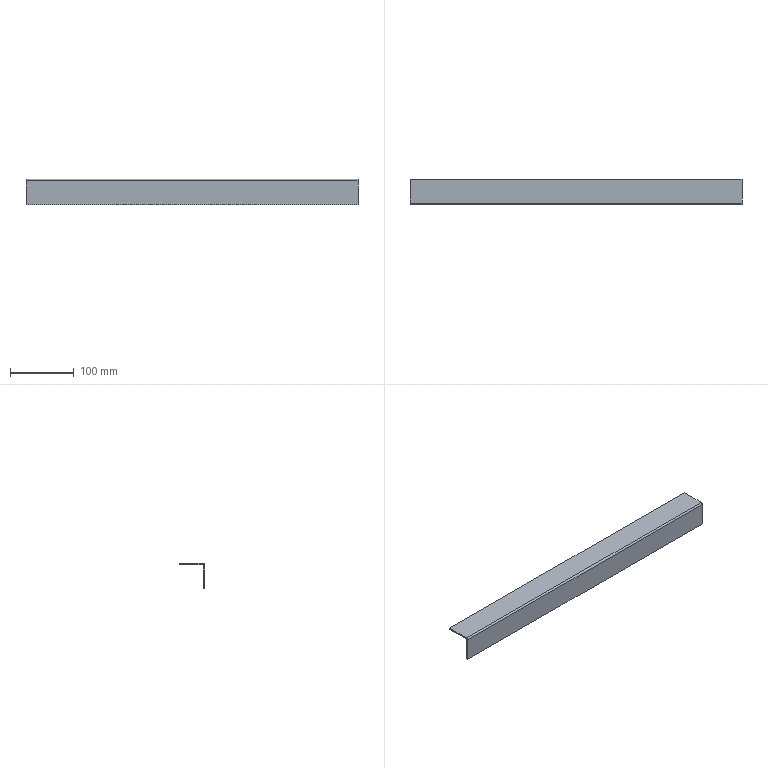Component | SolidWorks | BaseBracketAssembly-1_BaseBracketWidth-7 | 1 solid | 14 faces | box 520 x 40 x 40 mm | volume 80450 mm3 | plane 12 | cylinder 2 | commonest cylinder face diameters 5 x1 1 x1 | material 2.0mm Cold Rolled Plate
STEP:
#1=CARTESIAN_POINT('',(-11.983,-50.005,37.594));
#2=VERTEX_POINT('',#1);
#3=CARTESIAN_POINT('',(-11.983,-49.926,37.594));
#4=VERTEX_POINT('',#3);
#5=CARTESIAN_POINT('',(-11.983,-50.005,37.594));
#6=DIRECTION('',(0.,1.,0.));
#7=VECTOR('',#6,39.37);
#8=LINE('',#5,#7);
#9=EDGE_CURVE('',#2,#4,#8,.T.);
#10=ORIENTED_EDGE('',*,*,#9,.F.);
#11=CARTESIAN_POINT('',(-11.983,-49.907,37.692));
#12=VERTEX_POINT('',#11);
#13=CARTESIAN_POINT('',(-11.983,-49.907,37.594));
#14=DIRECTION('',(1.,-0.,-0.));
#15=DIRECTION('',(0.,1.,0.));
#16=AXIS2_PLACEMENT_3D('',#13,#14,#15);
#17=CIRCLE('',#16,0.09843);
#18=EDGE_CURVE('',#12,#2,#17,.T.);
#19=ORIENTED_EDGE('',*,*,#18,.F.);
#20=CARTESIAN_POINT('',(-11.983,-49.907,37.614));
#21=VERTEX_POINT('',#20);
#22=CARTESIAN_POINT('',(-11.983,-49.907,37.614));
#23=DIRECTION('',(0.,-0.,1.));
#24=VECTOR('',#23,39.37);
#25=LINE('',#22,#24);
#26=EDGE_CURVE('',#21,#12,#25,.T.);
#27=ORIENTED_EDGE('',*,*,#26,.F.);
#28=CARTESIAN_POINT('',(-11.983,-49.907,37.594));
#29=DIRECTION('',(1.,-0.,-0.));
#30=DIRECTION('',(0.,1.,0.));
#31=AXIS2_PLACEMENT_3D('',#28,#29,#30);
#32=CIRCLE('',#31,0.01969);
#33=EDGE_CURVE('',#21,#4,#32,.T.);
#34=ORIENTED_EDGE('',*,*,#33,.T.);
#35=EDGE_LOOP('',(#10,#19,#27,#34));
#36=FACE_OUTER_BOUND('',#35,.T.);
#37=CARTESIAN_POINT('',(-11.983,-50.005,37.594));
#38=DIRECTION('',(-1.,0.,0.));
#39=DIRECTION('',(0.,1.,0.));
#40=AXIS2_PLACEMENT_3D('',#37,#38,#39);
#41=PLANE('',#40);
#42=ADVANCED_FACE('',(#36),#41,.T.);
#43=CARTESIAN_POINT('',(-11.983,-50.005,36.118));
#44=VERTEX_POINT('',#43);
#45=CARTESIAN_POINT('',(-11.983,-50.005,36.118));
#46=DIRECTION('',(-0.,0.,-1.));
#47=VECTOR('',#46,39.37);
#48=LINE('',#45,#47);
#49=EDGE_CURVE('',#2,#44,#48,.T.);
#50=ORIENTED_EDGE('',*,*,#49,.F.);
#51=ORIENTED_EDGE('',*,*,#9,.T.);
#52=CARTESIAN_POINT('',(-11.983,-49.926,36.118));
#53=VERTEX_POINT('',#52);
#54=CARTESIAN_POINT('',(-11.983,-49.926,36.118));
#55=DIRECTION('',(-0.,0.,-1.));
#56=VECTOR('',#55,39.37);
#57=LINE('',#54,#56);
#58=EDGE_CURVE('',#4,#53,#57,.T.);
#59=ORIENTED_EDGE('',*,*,#58,.T.);
#60=CARTESIAN_POINT('',(-11.983,-50.005,36.118));
#61=DIRECTION('',(0.,1.,0.));
#62=VECTOR('',#61,39.37);
#63=LINE('',#60,#62);
#64=EDGE_CURVE('',#44,#53,#63,.T.);
#65=ORIENTED_EDGE('',*,*,#64,.F.);
#66=EDGE_LOOP('',(#50,#51,#59,#65));
#67=FACE_OUTER_BOUND('',#66,.T.);
#68=CARTESIAN_POINT('',(-11.983,-49.907,37.614));
#69=DIRECTION('',(-1.,0.,0.));
#70=DIRECTION('',(0.,1.,0.));
#71=AXIS2_PLACEMENT_3D('',#68,#69,#70);
#72=PLANE('',#71);
#73=ADVANCED_FACE('',(#67),#72,.T.);
#74=CARTESIAN_POINT('',(8.49,-49.907,37.692));
#75=VERTEX_POINT('',#74);
#76=CARTESIAN_POINT('',(8.49,-49.907,37.614));
#77=VERTEX_POINT('',#76);
#78=CARTESIAN_POINT('',(8.49,-49.907,37.692));
#79=DIRECTION('',(-0.,0.,-1.));
#80=VECTOR('',#79,39.37);
#81=LINE('',#78,#80);
#82=EDGE_CURVE('',#75,#77,#81,.T.);
#83=ORIENTED_EDGE('',*,*,#82,.F.);
#84=CARTESIAN_POINT('',(8.49,-50.005,37.594));
#85=VERTEX_POINT('',#84);
#86=CARTESIAN_POINT('',(8.49,-49.907,37.594));
#87=DIRECTION('',(1.,-0.,-0.));
#88=DIRECTION('',(0.,1.,0.));
#89=AXIS2_PLACEMENT_3D('',#86,#87,#88);
#90=CIRCLE('',#89,0.09843);
#91=EDGE_CURVE('',#75,#85,#90,.T.);
#92=ORIENTED_EDGE('',*,*,#91,.T.);
#93=CARTESIAN_POINT('',(8.49,-49.926,37.594));
#94=VERTEX_POINT('',#93);
#95=CARTESIAN_POINT('',(8.49,-49.926,37.594));
#96=DIRECTION('',(-0.,-1.,-0.));
#97=VECTOR('',#96,39.37);
#98=LINE('',#95,#97);
#99=EDGE_CURVE('',#94,#85,#98,.T.);
#100=ORIENTED_EDGE('',*,*,#99,.F.);
#101=CARTESIAN_POINT('',(8.49,-49.907,37.594));
#102=DIRECTION('',(1.,-0.,-0.));
#103=DIRECTION('',(0.,1.,0.));
#104=AXIS2_PLACEMENT_3D('',#101,#102,#103);
#105=CIRCLE('',#104,0.01969);
#106=EDGE_CURVE('',#77,#94,#105,.T.);
#107=ORIENTED_EDGE('',*,*,#106,.F.);
#108=EDGE_LOOP('',(#83,#92,#100,#107));
#109=FACE_OUTER_BOUND('',#108,.T.);
#110=CARTESIAN_POINT('',(8.49,-49.907,37.692));
#111=DIRECTION('',(1.,-0.,-0.));
#112=DIRECTION('',(-0.,-1.,-0.));
#113=AXIS2_PLACEMENT_3D('',#110,#111,#112);
#114=PLANE('',#113);
#115=ADVANCED_FACE('',(#109),#114,.T.);
#116=CARTESIAN_POINT('',(8.49,-48.43,37.692));
#117=VERTEX_POINT('',#116);
#118=CARTESIAN_POINT('',(8.49,-50.005,37.692));
#119=DIRECTION('',(-0.,-1.,-0.));
#120=VECTOR('',#119,39.37);
#121=LINE('',#118,#120);
#122=EDGE_CURVE('',#117,#75,#121,.T.);
#123=ORIENTED_EDGE('',*,*,#122,.T.);
#124=ORIENTED_EDGE('',*,*,#82,.T.);
#125=CARTESIAN_POINT('',(8.49,-48.43,37.614));
#126=VERTEX_POINT('',#125);
#127=CARTESIAN_POINT('',(8.49,-50.005,37.614));
#128=DIRECTION('',(-0.,-1.,-0.));
#129=VECTOR('',#128,39.37);
#130=LINE('',#127,#129);
#131=EDGE_CURVE('',#126,#77,#130,.T.);
#132=ORIENTED_EDGE('',*,*,#131,.F.);
#133=CARTESIAN_POINT('',(8.49,-48.43,37.614));
#134=DIRECTION('',(0.,-0.,1.));
#135=VECTOR('',#134,39.37);
#136=LINE('',#133,#135);
#137=EDGE_CURVE('',#126,#117,#136,.T.);
#138=ORIENTED_EDGE('',*,*,#137,.T.);
#139=EDGE_LOOP('',(#123,#124,#132,#138));
#140=FACE_OUTER_BOUND('',#139,.T.);
#141=CARTESIAN_POINT('',(8.49,-49.926,37.594));
#142=DIRECTION('',(1.,-0.,-0.));
#143=DIRECTION('',(-0.,-1.,-0.));
#144=AXIS2_PLACEMENT_3D('',#141,#142,#143);
#145=PLANE('',#144);
#146=ADVANCED_FACE('',(#140),#145,.T.);
#147=CARTESIAN_POINT('',(8.49,-49.926,36.118));
#148=VERTEX_POINT('',#147);
#149=CARTESIAN_POINT('',(8.49,-49.926,36.118));
#150=DIRECTION('',(-0.,0.,-1.));
#151=VECTOR('',#150,39.37);
#152=LINE('',#149,#151);
#153=EDGE_CURVE('',#94,#148,#152,.T.);
#154=ORIENTED_EDGE('',*,*,#153,.T.);
#155=CARTESIAN_POINT('',(-11.983,-49.926,36.118));
#156=DIRECTION('',(1.,-0.,-0.));
#157=VECTOR('',#156,39.37);
#158=LINE('',#155,#157);
#159=EDGE_CURVE('',#53,#148,#158,.T.);
#160=ORIENTED_EDGE('',*,*,#159,.F.);
#161=ORIENTED_EDGE('',*,*,#58,.F.);
#162=CARTESIAN_POINT('',(-11.983,-49.926,37.594));
#163=DIRECTION('',(1.,-0.,-0.));
#164=VECTOR('',#163,39.37);
#165=LINE('',#162,#164);
#166=EDGE_CURVE('',#4,#94,#165,.T.);
#167=ORIENTED_EDGE('',*,*,#166,.T.);
#168=EDGE_LOOP('',(#154,#160,#161,#167));
#169=FACE_OUTER_BOUND('',#168,.T.);
#170=CARTESIAN_POINT('',(-11.983,-49.926,36.118));
#171=DIRECTION('',(-0.,-1.,-0.));
#172=DIRECTION('',(-1.,0.,0.));
#173=AXIS2_PLACEMENT_3D('',#170,#171,#172);
#174=PLANE('',#173);
#175=ADVANCED_FACE('',(#169),#174,.F.);
#176=CARTESIAN_POINT('',(8.49,-50.005,36.118));
#177=VERTEX_POINT('',#176);
#178=CARTESIAN_POINT('',(8.49,-50.005,36.118));
#179=DIRECTION('',(0.,1.,0.));
#180=VECTOR('',#179,39.37);
#181=LINE('',#178,#180);
#182=EDGE_CURVE('',#177,#148,#181,.T.);
#183=ORIENTED_EDGE('',*,*,#182,.F.);
#184=CARTESIAN_POINT('',(-11.983,-50.005,36.118));
#185=DIRECTION('',(1.,-0.,-0.));
#186=VECTOR('',#185,39.37);
#187=LINE('',#184,#186);
#188=EDGE_CURVE('',#44,#177,#187,.T.);
#189=ORIENTED_EDGE('',*,*,#188,.F.);
#190=ORIENTED_EDGE('',*,*,#64,.T.);
#191=ORIENTED_EDGE('',*,*,#159,.T.);
#192=EDGE_LOOP('',(#183,#189,#190,#191));
#193=FACE_OUTER_BOUND('',#192,.T.);
#194=CARTESIAN_POINT('',(-11.983,-50.005,36.118));
#195=DIRECTION('',(-0.,0.,-1.));
#196=DIRECTION('',(-1.,0.,0.));
#197=AXIS2_PLACEMENT_3D('',#194,#195,#196);
#198=PLANE('',#197);
#199=ADVANCED_FACE('',(#193),#198,.T.);
#200=CARTESIAN_POINT('',(8.49,-50.005,36.118));
#201=DIRECTION('',(-0.,0.,-1.));
#202=VECTOR('',#201,39.37);
#203=LINE('',#200,#202);
#204=EDGE_CURVE('',#85,#177,#203,.T.);
#205=ORIENTED_EDGE('',*,*,#204,.F.);
#206=CARTESIAN_POINT('',(-11.983,-50.005,37.594));
#207=DIRECTION('',(1.,-0.,-0.));
#208=VECTOR('',#207,39.37);
#209=LINE('',#206,#208);
#210=EDGE_CURVE('',#2,#85,#209,.T.);
#211=ORIENTED_EDGE('',*,*,#210,.F.);
#212=ORIENTED_EDGE('',*,*,#49,.T.);
#213=ORIENTED_EDGE('',*,*,#188,.T.);
#214=EDGE_LOOP('',(#205,#211,#212,#213));
#215=FACE_OUTER_BOUND('',#214,.T.);
#216=CARTESIAN_POINT('',(-11.983,-50.005,36.118));
#217=DIRECTION('',(-0.,-1.,-0.));
#218=DIRECTION('',(-1.,0.,0.));
#219=AXIS2_PLACEMENT_3D('',#216,#217,#218);
#220=PLANE('',#219);
#221=ADVANCED_FACE('',(#215),#220,.T.);
#222=ORIENTED_EDGE('',*,*,#91,.F.);
#223=CARTESIAN_POINT('',(-11.983,-49.907,37.692));
#224=DIRECTION('',(1.,-0.,-0.));
#225=VECTOR('',#224,39.37);
#226=LINE('',#223,#225);
#227=EDGE_CURVE('',#12,#75,#226,.T.);
#228=ORIENTED_EDGE('',*,*,#227,.F.);
#229=ORIENTED_EDGE('',*,*,#18,.T.);
#230=ORIENTED_EDGE('',*,*,#210,.T.);
#231=EDGE_LOOP('',(#222,#228,#229,#230));
#232=FACE_OUTER_BOUND('',#231,.T.);
#233=CARTESIAN_POINT('',(-11.983,-49.907,37.594));
#234=DIRECTION('',(1.,-0.,-0.));
#235=DIRECTION('',(0.,-1.,0.));
#236=AXIS2_PLACEMENT_3D('',#233,#234,#235);
#237=CYLINDRICAL_SURFACE('',#236,0.09843);
#238=ADVANCED_FACE('',(#232),#237,.T.);
#239=ORIENTED_EDGE('',*,*,#122,.F.);
#240=CARTESIAN_POINT('',(-11.983,-48.43,37.692));
#241=VERTEX_POINT('',#240);
#242=CARTESIAN_POINT('',(-11.983,-48.43,37.692));
#243=DIRECTION('',(1.,-0.,-0.));
#244=VECTOR('',#243,39.37);
#245=LINE('',#242,#244);
#246=EDGE_CURVE('',#241,#117,#245,.T.);
#247=ORIENTED_EDGE('',*,*,#246,.F.);
#248=CARTESIAN_POINT('',(-11.983,-50.005,37.692));
#249=DIRECTION('',(-0.,-1.,-0.));
#250=VECTOR('',#249,39.37);
#251=LINE('',#248,#250);
#252=EDGE_CURVE('',#241,#12,#251,.T.);
#253=ORIENTED_EDGE('',*,*,#252,.T.);
#254=ORIENTED_EDGE('',*,*,#227,.T.);
#255=EDGE_LOOP('',(#239,#247,#253,#254));
#256=FACE_OUTER_BOUND('',#255,.T.);
#257=CARTESIAN_POINT('',(-11.983,-50.005,37.692));
#258=DIRECTION('',(0.,-0.,1.));
#259=DIRECTION('',(1.,-0.,-0.));
#260=AXIS2_PLACEMENT_3D('',#257,#258,#259);
#261=PLANE('',#260);
#262=ADVANCED_FACE('',(#256),#261,.T.);
#263=ORIENTED_EDGE('',*,*,#137,.F.);
#264=CARTESIAN_POINT('',(-11.983,-48.43,37.614));
#265=VERTEX_POINT('',#264);
#266=CARTESIAN_POINT('',(-11.983,-48.43,37.614));
#267=DIRECTION('',(1.,-0.,-0.));
#268=VECTOR('',#267,39.37);
#269=LINE('',#266,#268);
#270=EDGE_CURVE('',#265,#126,#269,.T.);
#271=ORIENTED_EDGE('',*,*,#270,.F.);
#272=CARTESIAN_POINT('',(-11.983,-48.43,37.614));
#273=DIRECTION('',(0.,-0.,1.));
#274=VECTOR('',#273,39.37);
#275=LINE('',#272,#274);
#276=EDGE_CURVE('',#265,#241,#275,.T.);
#277=ORIENTED_EDGE('',*,*,#276,.T.);
#278=ORIENTED_EDGE('',*,*,#246,.T.);
#279=EDGE_LOOP('',(#263,#271,#277,#278));
#280=FACE_OUTER_BOUND('',#279,.T.);
#281=CARTESIAN_POINT('',(-11.983,-48.43,37.614));
#282=DIRECTION('',(0.,1.,0.));
#283=DIRECTION('',(1.,-0.,-0.));
#284=AXIS2_PLACEMENT_3D('',#281,#282,#283);
#285=PLANE('',#284);
#286=ADVANCED_FACE('',(#280),#285,.T.);
#287=ORIENTED_EDGE('',*,*,#131,.T.);
#288=CARTESIAN_POINT('',(-11.983,-49.907,37.614));
#289=DIRECTION('',(1.,-0.,-0.));
#290=VECTOR('',#289,39.37);
#291=LINE('',#288,#290);
#292=EDGE_CURVE('',#21,#77,#291,.T.);
#293=ORIENTED_EDGE('',*,*,#292,.F.);
#294=CARTESIAN_POINT('',(-11.983,-50.005,37.614));
#295=DIRECTION('',(-0.,-1.,-0.));
#296=VECTOR('',#295,39.37);
#297=LINE('',#294,#296);
#298=EDGE_CURVE('',#265,#21,#297,.T.);
#299=ORIENTED_EDGE('',*,*,#298,.F.);
#300=ORIENTED_EDGE('',*,*,#270,.T.);
#301=EDGE_LOOP('',(#287,#293,#299,#300));
#302=FACE_OUTER_BOUND('',#301,.T.);
#303=CARTESIAN_POINT('',(-11.983,-50.005,37.614));
#304=DIRECTION('',(0.,-0.,1.));
#305=DIRECTION('',(1.,-0.,-0.));
#306=AXIS2_PLACEMENT_3D('',#303,#304,#305);
#307=PLANE('',#306);
#308=ADVANCED_FACE('',(#302),#307,.F.);
#309=ORIENTED_EDGE('',*,*,#106,.T.);
#310=ORIENTED_EDGE('',*,*,#166,.F.);
#311=ORIENTED_EDGE('',*,*,#33,.F.);
#312=ORIENTED_EDGE('',*,*,#292,.T.);
#313=EDGE_LOOP('',(#309,#310,#311,#312));
#314=FACE_OUTER_BOUND('',#313,.T.);
#315=CARTESIAN_POINT('',(-11.983,-49.907,37.594));
#316=DIRECTION('',(1.,-0.,-0.));
#317=DIRECTION('',(0.,-1.,0.));
#318=AXIS2_PLACEMENT_3D('',#315,#316,#317);
#319=CYLINDRICAL_SURFACE('',#318,0.01969);
#320=ADVANCED_FACE('',(#314),#319,.F.);
#321=ORIENTED_EDGE('',*,*,#298,.T.);
#322=ORIENTED_EDGE('',*,*,#26,.T.);
#323=ORIENTED_EDGE('',*,*,#252,.F.);
#324=ORIENTED_EDGE('',*,*,#276,.F.);
#325=EDGE_LOOP('',(#321,#322,#323,#324));
#326=FACE_OUTER_BOUND('',#325,.T.);
#327=CARTESIAN_POINT('',(-11.983,-49.907,37.594));
#328=DIRECTION('',(-1.,0.,0.));
#329=DIRECTION('',(0.,1.,0.));
#330=AXIS2_PLACEMENT_3D('',#327,#328,#329);
#331=PLANE('',#330);
#332=ADVANCED_FACE('',(#326),#331,.T.);
#333=ORIENTED_EDGE('',*,*,#153,.F.);
#334=ORIENTED_EDGE('',*,*,#99,.T.);
#335=ORIENTED_EDGE('',*,*,#204,.T.);
#336=ORIENTED_EDGE('',*,*,#182,.T.);
#337=EDGE_LOOP('',(#333,#334,#335,#336));
#338=FACE_OUTER_BOUND('',#337,.T.);
#339=CARTESIAN_POINT('',(8.49,-49.907,37.594));
#340=DIRECTION('',(-1.,0.,0.));
#341=DIRECTION('',(0.,1.,0.));
#342=AXIS2_PLACEMENT_3D('',#339,#340,#341);
#343=PLANE('',#342);
#344=ADVANCED_FACE('',(#338),#343,.F.);
#345=CLOSED_SHELL('',(#42,#73,#115,#146,#175,#199,#221,#238,#262,#286,#308,#320,#332,#344));
#346=MANIFOLD_SOLID_BREP('',#345);
#347=CARTESIAN_POINT('',(0.,0.,0.));
#348=DIRECTION('',(0.,0.,1.));
#349=DIRECTION('',(1.,0.,0.));
#350=AXIS2_PLACEMENT_3D('',#347,#348,#349);
#351=(LENGTH_UNIT()NAMED_UNIT(*)SI_UNIT($,.METRE.));
#352=LENGTH_MEASURE_WITH_UNIT(LENGTH_MEASURE(0.0254),#351);
#353=DIMENSIONAL_EXPONENTS(1.,0.,0.,0.,0.,0.,0.);
#354=(CONVERSION_BASED_UNIT('',#352)LENGTH_UNIT()NAMED_UNIT(#353));
#355=UNCERTAINTY_MEASURE_WITH_UNIT(LENGTH_MEASURE(0.00001),#354,'','');
#356=(NAMED_UNIT(*)PLANE_ANGLE_UNIT()SI_UNIT($,.RADIAN.));
#357=(NAMED_UNIT(*)SI_UNIT($,.STERADIAN.)SOLID_ANGLE_UNIT());
#358=(GEOMETRIC_REPRESENTATION_CONTEXT(3)GLOBAL_UNCERTAINTY_ASSIGNED_CONTEXT((#355))GLOBAL_UNIT_ASSIGNED_CONTEXT((#354,#356,#357))REPRESENTATION_CONTEXT('',''));
#359=ADVANCED_BREP_SHAPE_REPRESENTATION('',(#346,#350),#358);
#360=COLOUR_RGB('',0.7922,0.8196,0.9333);
#361=FILL_AREA_STYLE_COLOUR('',#360);
#362=FILL_AREA_STYLE('',(#361));
#363=SURFACE_STYLE_FILL_AREA(#362);
#364=SURFACE_SIDE_STYLE('',(#363));
#365=SURFACE_STYLE_USAGE(.BOTH.,#364);
#366=PRESENTATION_STYLE_ASSIGNMENT((#365));
#367=STYLED_ITEM('',(#366),#346);
#368=(LENGTH_UNIT()NAMED_UNIT(*)SI_UNIT($,.METRE.));
#369=LENGTH_MEASURE_WITH_UNIT(LENGTH_MEASURE(0.0254),#368);
#370=DIMENSIONAL_EXPONENTS(1.,0.,0.,0.,0.,0.,0.);
#371=(CONVERSION_BASED_UNIT('',#369)LENGTH_UNIT()NAMED_UNIT(#370));
#372=UNCERTAINTY_MEASURE_WITH_UNIT(LENGTH_MEASURE(0.00001),#371,'','');
#373=(NAMED_UNIT(*)PLANE_ANGLE_UNIT()SI_UNIT($,.RADIAN.));
#374=(NAMED_UNIT(*)SI_UNIT($,.STERADIAN.)SOLID_ANGLE_UNIT());
#375=(GEOMETRIC_REPRESENTATION_CONTEXT(3)GLOBAL_UNCERTAINTY_ASSIGNED_CONTEXT((#372))GLOBAL_UNIT_ASSIGNED_CONTEXT((#371,#373,#374))REPRESENTATION_CONTEXT('',''));
#376=MECHANICAL_DESIGN_GEOMETRIC_PRESENTATION_REPRESENTATION('',(#367),#375);
#377=PRESENTATION_LAYER_ASSIGNMENT('','',(#367));